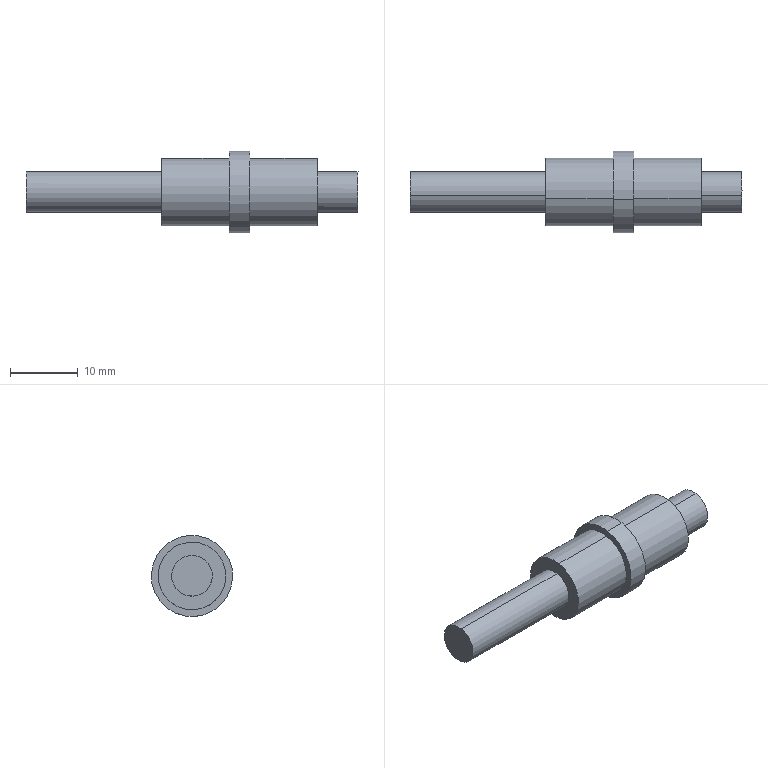Component | SolidWorks | GrippingMandrel-1 | 1 solid | 16 faces | box 49.01 x 12 x 12 mm | volume 2645 mm3 | cylinder 10 | plane 6 | commonest cylinder face diameters 6 x4 10 x4 12 x2
build123d program:
from build123d import *

# Parameters (mm, degrees)
SKETCH1_R           = 5
BOSS_EXTRUDE1_DEPTH = 10
SKETCH2_R           = 3
BOSS_EXTRUDE2_DEPTH = 6
SKETCH4_R           = 6
BOSS_EXTRUDE4_DEPTH = 3
SKETCH5_R           = 5
BOSS_EXTRUDE5_DEPTH = 10
BOSS_EXTRUDE6_START = 20
SKETCH6_R           = 3
BOSS_EXTRUDE6_DEPTH = 20


with BuildPart() as part:
    # Sketch1 → Boss-Extrude1 (new body)
    with BuildSketch(Plane(origin=(0, 0, 0), x_dir=(1, 0, 0), z_dir=(0, 1, 0))):
        with Locations(Location((0, 0, 0), (0, 0, 270))):
            Circle(SKETCH1_R)
    extrude(amount=BOSS_EXTRUDE1_DEPTH)

    # Sketch2 → Boss-Extrude2 (add)
    with BuildSketch(Plane(origin=(0, 0, 0), x_dir=(-1, 0, 0), z_dir=(0, -1, 0))):
        with Locations(Location((0, 0, 0), (0, 0, 90))):
            Circle(SKETCH2_R)
    extrude(amount=BOSS_EXTRUDE2_DEPTH)

    # Sketch4 → Boss-Extrude4 (add)
    with BuildSketch(Plane(origin=(0, 10, 0), x_dir=(1, 0, 0), z_dir=(0, 1, 0))):
        with Locations(Location((0, 0, 0), (0, 0, 270))):
            Circle(SKETCH4_R)
    extrude(amount=BOSS_EXTRUDE4_DEPTH)

    # Sketch5 → Boss-Extrude5 (add)
    with BuildSketch(Plane(origin=(0, 13, 0), x_dir=(1, 0, 0), z_dir=(0, 1, 0))):
        with Locations(Location((0, 0, 0), (0, 0, 270))):
            Circle(SKETCH5_R)
    extrude(amount=BOSS_EXTRUDE5_DEPTH)

    # Sketch6 → Boss-Extrude6 (add)
    with BuildSketch(Plane(origin=(0, 23, 0), x_dir=(1, 0, 0), z_dir=(0, 1, 0)).offset(BOSS_EXTRUDE6_START)):
        with Locations(Location((0, 0, 0), (0, 0, 90))):
            Circle(SKETCH6_R)
    extrude(amount=-BOSS_EXTRUDE6_DEPTH)


solid = part.part

# Placed as in the assembly
solid = solid.moved(Location((-104.642, 765.309, 1092.206), (-22.496, 0.05719, 90.024)))
STEP:
#1=CARTESIAN_POINT('',(-5.813,30.109,43.118));
#2=VERTEX_POINT('',#1);
#3=CARTESIAN_POINT('',(-5.813,30.152,42.886));
#4=VERTEX_POINT('',#3);
#5=CARTESIAN_POINT('',(-5.813,30.13,43.002));
#6=DIRECTION('',(-1.,-0.,0.00108));
#7=DIRECTION('',(0.001062,-0.1828,0.9831));
#8=AXIS2_PLACEMENT_3D('',#5,#6,#7);
#9=CIRCLE('',#8,0.1181);
#10=EDGE_CURVE('',#2,#4,#9,.T.);
#11=ORIENTED_EDGE('',*,*,#10,.F.);
#12=CARTESIAN_POINT('',(-5.025,30.109,43.117));
#13=VERTEX_POINT('',#12);
#14=CARTESIAN_POINT('',(-5.813,30.109,43.118));
#15=DIRECTION('',(1.,0.,-0.00108));
#16=VECTOR('',#15,39.37);
#17=LINE('',#14,#16);
#18=EDGE_CURVE('',#2,#13,#17,.T.);
#19=ORIENTED_EDGE('',*,*,#18,.T.);
#20=CARTESIAN_POINT('',(-5.025,30.152,42.885));
#21=VERTEX_POINT('',#20);
#22=CARTESIAN_POINT('',(-5.025,30.13,43.001));
#23=DIRECTION('',(-1.,-0.,0.00108));
#24=DIRECTION('',(0.001062,-0.1828,0.9831));
#25=AXIS2_PLACEMENT_3D('',#22,#23,#24);
#26=CIRCLE('',#25,0.1181);
#27=EDGE_CURVE('',#13,#21,#26,.T.);
#28=ORIENTED_EDGE('',*,*,#27,.T.);
#29=CARTESIAN_POINT('',(-5.813,30.152,42.886));
#30=DIRECTION('',(1.,0.,-0.00108));
#31=VECTOR('',#30,39.37);
#32=LINE('',#29,#31);
#33=EDGE_CURVE('',#4,#21,#32,.T.);
#34=ORIENTED_EDGE('',*,*,#33,.F.);
#35=EDGE_LOOP('',(#11,#19,#28,#34));
#36=FACE_OUTER_BOUND('',#35,.T.);
#37=CARTESIAN_POINT('',(-5.813,30.13,43.002));
#38=DIRECTION('',(1.,0.,-0.00108));
#39=DIRECTION('',(-0.001062,0.1828,-0.9831));
#40=AXIS2_PLACEMENT_3D('',#37,#38,#39);
#41=CYLINDRICAL_SURFACE('',#40,0.1181);
#42=ADVANCED_FACE('',(#36),#41,.T.);
#43=CARTESIAN_POINT('',(-5.025,30.094,43.195));
#44=VERTEX_POINT('',#43);
#45=CARTESIAN_POINT('',(-5.025,30.166,42.808));
#46=VERTEX_POINT('',#45);
#47=CARTESIAN_POINT('',(-5.025,30.13,43.001));
#48=DIRECTION('',(-1.,-0.,0.00108));
#49=DIRECTION('',(0.001062,-0.1828,0.9831));
#50=AXIS2_PLACEMENT_3D('',#47,#48,#49);
#51=CIRCLE('',#50,0.1969);
#52=EDGE_CURVE('',#44,#46,#51,.T.);
#53=ORIENTED_EDGE('',*,*,#52,.F.);
#54=CARTESIAN_POINT('',(-4.631,30.094,43.194));
#55=VERTEX_POINT('',#54);
#56=CARTESIAN_POINT('',(-5.025,30.094,43.195));
#57=DIRECTION('',(1.,0.,-0.00108));
#58=VECTOR('',#57,39.37);
#59=LINE('',#56,#58);
#60=EDGE_CURVE('',#44,#55,#59,.T.);
#61=ORIENTED_EDGE('',*,*,#60,.T.);
#62=CARTESIAN_POINT('',(-4.632,30.166,42.807));
#63=VERTEX_POINT('',#62);
#64=CARTESIAN_POINT('',(-4.632,30.13,43.001));
#65=DIRECTION('',(-1.,-0.,0.00108));
#66=DIRECTION('',(0.001062,-0.1828,0.9831));
#67=AXIS2_PLACEMENT_3D('',#64,#65,#66);
#68=CIRCLE('',#67,0.1969);
#69=EDGE_CURVE('',#55,#63,#68,.T.);
#70=ORIENTED_EDGE('',*,*,#69,.T.);
#71=CARTESIAN_POINT('',(-5.025,30.166,42.808));
#72=DIRECTION('',(1.,0.,-0.00108));
#73=VECTOR('',#72,39.37);
#74=LINE('',#71,#73);
#75=EDGE_CURVE('',#46,#63,#74,.T.);
#76=ORIENTED_EDGE('',*,*,#75,.F.);
#77=EDGE_LOOP('',(#53,#61,#70,#76));
#78=FACE_OUTER_BOUND('',#77,.T.);
#79=CARTESIAN_POINT('',(-5.025,30.13,43.001));
#80=DIRECTION('',(1.,0.,-0.00108));
#81=DIRECTION('',(-0.001062,0.1828,-0.9831));
#82=AXIS2_PLACEMENT_3D('',#79,#80,#81);
#83=CYLINDRICAL_SURFACE('',#82,0.1969);
#84=ADVANCED_FACE('',(#78),#83,.T.);
#85=CARTESIAN_POINT('',(-4.631,30.087,43.233));
#86=VERTEX_POINT('',#85);
#87=CARTESIAN_POINT('',(-4.632,30.173,42.769));
#88=VERTEX_POINT('',#87);
#89=CARTESIAN_POINT('',(-4.632,30.13,43.001));
#90=DIRECTION('',(-1.,-0.,0.00108));
#91=DIRECTION('',(0.001062,-0.1828,0.9831));
#92=AXIS2_PLACEMENT_3D('',#89,#90,#91);
#93=CIRCLE('',#92,0.2362);
#94=EDGE_CURVE('',#86,#88,#93,.T.);
#95=ORIENTED_EDGE('',*,*,#94,.F.);
#96=CARTESIAN_POINT('',(-4.513,30.087,43.233));
#97=VERTEX_POINT('',#96);
#98=CARTESIAN_POINT('',(-4.631,30.087,43.233));
#99=DIRECTION('',(1.,0.,-0.00108));
#100=VECTOR('',#99,39.37);
#101=LINE('',#98,#100);
#102=EDGE_CURVE('',#86,#97,#101,.T.);
#103=ORIENTED_EDGE('',*,*,#102,.T.);
#104=CARTESIAN_POINT('',(-4.514,30.173,42.768));
#105=VERTEX_POINT('',#104);
#106=CARTESIAN_POINT('',(-4.513,30.13,43.001));
#107=DIRECTION('',(-1.,-0.,0.00108));
#108=DIRECTION('',(0.001062,-0.1828,0.9831));
#109=AXIS2_PLACEMENT_3D('',#106,#107,#108);
#110=CIRCLE('',#109,0.2362);
#111=EDGE_CURVE('',#97,#105,#110,.T.);
#112=ORIENTED_EDGE('',*,*,#111,.T.);
#113=CARTESIAN_POINT('',(-4.632,30.173,42.769));
#114=DIRECTION('',(1.,0.,-0.00108));
#115=VECTOR('',#114,39.37);
#116=LINE('',#113,#115);
#117=EDGE_CURVE('',#88,#105,#116,.T.);
#118=ORIENTED_EDGE('',*,*,#117,.F.);
#119=EDGE_LOOP('',(#95,#103,#112,#118));
#120=FACE_OUTER_BOUND('',#119,.T.);
#121=CARTESIAN_POINT('',(-4.632,30.13,43.001));
#122=DIRECTION('',(1.,0.,-0.00108));
#123=DIRECTION('',(-0.001062,0.1828,-0.9831));
#124=AXIS2_PLACEMENT_3D('',#121,#122,#123);
#125=CYLINDRICAL_SURFACE('',#124,0.2362);
#126=ADVANCED_FACE('',(#120),#125,.T.);
#127=CARTESIAN_POINT('',(-3.884,30.152,42.884));
#128=VERTEX_POINT('',#127);
#129=CARTESIAN_POINT('',(-3.883,30.109,43.116));
#130=VERTEX_POINT('',#129);
#131=CARTESIAN_POINT('',(-3.884,30.13,43.));
#132=DIRECTION('',(1.,0.,-0.00108));
#133=DIRECTION('',(-0.001062,0.1828,-0.9831));
#134=AXIS2_PLACEMENT_3D('',#131,#132,#133);
#135=CIRCLE('',#134,0.1181);
#136=EDGE_CURVE('',#128,#130,#135,.T.);
#137=ORIENTED_EDGE('',*,*,#136,.F.);
#138=CARTESIAN_POINT('',(-4.12,30.152,42.884));
#139=VERTEX_POINT('',#138);
#140=CARTESIAN_POINT('',(-3.884,30.152,42.884));
#141=DIRECTION('',(-1.,-0.,0.00108));
#142=VECTOR('',#141,39.37);
#143=LINE('',#140,#142);
#144=EDGE_CURVE('',#128,#139,#143,.T.);
#145=ORIENTED_EDGE('',*,*,#144,.T.);
#146=CARTESIAN_POINT('',(-4.12,30.109,43.116));
#147=VERTEX_POINT('',#146);
#148=CARTESIAN_POINT('',(-4.12,30.13,43.));
#149=DIRECTION('',(1.,0.,-0.00108));
#150=DIRECTION('',(-0.001062,0.1828,-0.9831));
#151=AXIS2_PLACEMENT_3D('',#148,#149,#150);
#152=CIRCLE('',#151,0.1181);
#153=EDGE_CURVE('',#139,#147,#152,.T.);
#154=ORIENTED_EDGE('',*,*,#153,.T.);
#155=CARTESIAN_POINT('',(-3.883,30.109,43.116));
#156=DIRECTION('',(-1.,-0.,0.00108));
#157=VECTOR('',#156,39.37);
#158=LINE('',#155,#157);
#159=EDGE_CURVE('',#130,#147,#158,.T.);
#160=ORIENTED_EDGE('',*,*,#159,.F.);
#161=EDGE_LOOP('',(#137,#145,#154,#160));
#162=FACE_OUTER_BOUND('',#161,.T.);
#163=CARTESIAN_POINT('',(-3.884,30.13,43.));
#164=DIRECTION('',(-1.,-0.,0.00108));
#165=DIRECTION('',(0.001062,-0.1828,0.9831));
#166=AXIS2_PLACEMENT_3D('',#163,#164,#165);
#167=CYLINDRICAL_SURFACE('',#166,0.1181);
#168=ADVANCED_FACE('',(#162),#167,.T.);
#169=CARTESIAN_POINT('',(-4.513,30.094,43.194));
#170=VERTEX_POINT('',#169);
#171=CARTESIAN_POINT('',(-4.514,30.166,42.807));
#172=VERTEX_POINT('',#171);
#173=CARTESIAN_POINT('',(-4.513,30.13,43.001));
#174=DIRECTION('',(-1.,-0.,0.00108));
#175=DIRECTION('',(0.001062,-0.1828,0.9831));
#176=AXIS2_PLACEMENT_3D('',#173,#174,#175);
#177=CIRCLE('',#176,0.1969);
#178=EDGE_CURVE('',#170,#172,#177,.T.);
#179=ORIENTED_EDGE('',*,*,#178,.F.);
#180=CARTESIAN_POINT('',(-4.12,30.094,43.194));
#181=VERTEX_POINT('',#180);
#182=CARTESIAN_POINT('',(-4.513,30.094,43.194));
#183=DIRECTION('',(1.,0.,-0.00108));
#184=VECTOR('',#183,39.37);
#185=LINE('',#182,#184);
#186=EDGE_CURVE('',#170,#181,#185,.T.);
#187=ORIENTED_EDGE('',*,*,#186,.T.);
#188=CARTESIAN_POINT('',(-4.12,30.166,42.807));
#189=VERTEX_POINT('',#188);
#190=CARTESIAN_POINT('',(-4.12,30.13,43.));
#191=DIRECTION('',(-1.,-0.,0.00108));
#192=DIRECTION('',(0.001062,-0.1828,0.9831));
#193=AXIS2_PLACEMENT_3D('',#190,#191,#192);
#194=CIRCLE('',#193,0.1969);
#195=EDGE_CURVE('',#181,#189,#194,.T.);
#196=ORIENTED_EDGE('',*,*,#195,.T.);
#197=CARTESIAN_POINT('',(-4.514,30.166,42.807));
#198=DIRECTION('',(1.,0.,-0.00108));
#199=VECTOR('',#198,39.37);
#200=LINE('',#197,#199);
#201=EDGE_CURVE('',#172,#189,#200,.T.);
#202=ORIENTED_EDGE('',*,*,#201,.F.);
#203=EDGE_LOOP('',(#179,#187,#196,#202));
#204=FACE_OUTER_BOUND('',#203,.T.);
#205=CARTESIAN_POINT('',(-4.513,30.13,43.001));
#206=DIRECTION('',(1.,0.,-0.00108));
#207=DIRECTION('',(-0.001062,0.1828,-0.9831));
#208=AXIS2_PLACEMENT_3D('',#205,#206,#207);
#209=CYLINDRICAL_SURFACE('',#208,0.1969);
#210=ADVANCED_FACE('',(#204),#209,.T.);
#211=ORIENTED_EDGE('',*,*,#186,.F.);
#212=CARTESIAN_POINT('',(-4.513,30.13,43.001));
#213=DIRECTION('',(-1.,-0.,0.00108));
#214=DIRECTION('',(0.001062,-0.1828,0.9831));
#215=AXIS2_PLACEMENT_3D('',#212,#213,#214);
#216=CIRCLE('',#215,0.1969);
#217=EDGE_CURVE('',#172,#170,#216,.T.);
#218=ORIENTED_EDGE('',*,*,#217,.F.);
#219=ORIENTED_EDGE('',*,*,#201,.T.);
#220=CARTESIAN_POINT('',(-4.12,30.13,43.));
#221=DIRECTION('',(-1.,-0.,0.00108));
#222=DIRECTION('',(0.001062,-0.1828,0.9831));
#223=AXIS2_PLACEMENT_3D('',#220,#221,#222);
#224=CIRCLE('',#223,0.1969);
#225=EDGE_CURVE('',#189,#181,#224,.T.);
#226=ORIENTED_EDGE('',*,*,#225,.T.);
#227=EDGE_LOOP('',(#211,#218,#219,#226));
#228=FACE_OUTER_BOUND('',#227,.T.);
#229=CARTESIAN_POINT('',(-4.513,30.13,43.001));
#230=DIRECTION('',(1.,0.,-0.00108));
#231=DIRECTION('',(-0.001062,0.1828,-0.9831));
#232=AXIS2_PLACEMENT_3D('',#229,#230,#231);
#233=CYLINDRICAL_SURFACE('',#232,0.1969);
#234=ADVANCED_FACE('',(#228),#233,.T.);
#235=CARTESIAN_POINT('',(-4.12,30.13,43.));
#236=DIRECTION('',(1.,0.,-0.00108));
#237=DIRECTION('',(-0.001062,0.1828,-0.9831));
#238=AXIS2_PLACEMENT_3D('',#235,#236,#237);
#239=CIRCLE('',#238,0.1181);
#240=EDGE_CURVE('',#147,#139,#239,.T.);
#241=ORIENTED_EDGE('',*,*,#240,.F.);
#242=ORIENTED_EDGE('',*,*,#153,.F.);
#243=EDGE_LOOP('',(#241,#242));
#244=FACE_BOUND('',#243,.T.);
#245=ORIENTED_EDGE('',*,*,#225,.F.);
#246=ORIENTED_EDGE('',*,*,#195,.F.);
#247=EDGE_LOOP('',(#245,#246));
#248=FACE_OUTER_BOUND('',#247,.T.);
#249=CARTESIAN_POINT('',(-4.12,30.13,43.));
#250=DIRECTION('',(-1.,-0.,0.00108));
#251=DIRECTION('',(0.001062,-0.1828,0.9831));
#252=AXIS2_PLACEMENT_3D('',#249,#250,#251);
#253=PLANE('',#252);
#254=ADVANCED_FACE('',(#244,#248),#253,.F.);
#255=ORIENTED_EDGE('',*,*,#144,.F.);
#256=CARTESIAN_POINT('',(-3.884,30.13,43.));
#257=DIRECTION('',(1.,0.,-0.00108));
#258=DIRECTION('',(-0.001062,0.1828,-0.9831));
#259=AXIS2_PLACEMENT_3D('',#256,#257,#258);
#260=CIRCLE('',#259,0.1181);
#261=EDGE_CURVE('',#130,#128,#260,.T.);
#262=ORIENTED_EDGE('',*,*,#261,.F.);
#263=ORIENTED_EDGE('',*,*,#159,.T.);
#264=ORIENTED_EDGE('',*,*,#240,.T.);
#265=EDGE_LOOP('',(#255,#262,#263,#264));
#266=FACE_OUTER_BOUND('',#265,.T.);
#267=CARTESIAN_POINT('',(-3.884,30.13,43.));
#268=DIRECTION('',(-1.,-0.,0.00108));
#269=DIRECTION('',(0.001062,-0.1828,0.9831));
#270=AXIS2_PLACEMENT_3D('',#267,#268,#269);
#271=CYLINDRICAL_SURFACE('',#270,0.1181);
#272=ADVANCED_FACE('',(#266),#271,.T.);
#273=ORIENTED_EDGE('',*,*,#261,.T.);
#274=ORIENTED_EDGE('',*,*,#136,.T.);
#275=EDGE_LOOP('',(#273,#274));
#276=FACE_OUTER_BOUND('',#275,.T.);
#277=CARTESIAN_POINT('',(-3.884,30.13,43.));
#278=DIRECTION('',(1.,0.,-0.00108));
#279=DIRECTION('',(-0.001062,0.1828,-0.9831));
#280=AXIS2_PLACEMENT_3D('',#277,#278,#279);
#281=PLANE('',#280);
#282=ADVANCED_FACE('',(#276),#281,.T.);
#283=ORIENTED_EDGE('',*,*,#102,.F.);
#284=CARTESIAN_POINT('',(-4.632,30.13,43.001));
#285=DIRECTION('',(-1.,-0.,0.00108));
#286=DIRECTION('',(0.001062,-0.1828,0.9831));
#287=AXIS2_PLACEMENT_3D('',#284,#285,#286);
#288=CIRCLE('',#287,0.2362);
#289=EDGE_CURVE('',#88,#86,#288,.T.);
#290=ORIENTED_EDGE('',*,*,#289,.F.);
#291=ORIENTED_EDGE('',*,*,#117,.T.);
#292=CARTESIAN_POINT('',(-4.513,30.13,43.001));
#293=DIRECTION('',(-1.,-0.,0.00108));
#294=DIRECTION('',(0.001062,-0.1828,0.9831));
#295=AXIS2_PLACEMENT_3D('',#292,#293,#294);
#296=CIRCLE('',#295,0.2362);
#297=EDGE_CURVE('',#105,#97,#296,.T.);
#298=ORIENTED_EDGE('',*,*,#297,.T.);
#299=EDGE_LOOP('',(#283,#290,#291,#298));
#300=FACE_OUTER_BOUND('',#299,.T.);
#301=CARTESIAN_POINT('',(-4.632,30.13,43.001));
#302=DIRECTION('',(1.,0.,-0.00108));
#303=DIRECTION('',(-0.001062,0.1828,-0.9831));
#304=AXIS2_PLACEMENT_3D('',#301,#302,#303);
#305=CYLINDRICAL_SURFACE('',#304,0.2362);
#306=ADVANCED_FACE('',(#300),#305,.T.);
#307=CARTESIAN_POINT('',(-4.632,30.13,43.001));
#308=DIRECTION('',(-1.,-0.,0.00108));
#309=DIRECTION('',(0.001062,-0.1828,0.9831));
#310=AXIS2_PLACEMENT_3D('',#307,#308,#309);
#311=CIRCLE('',#310,0.1969);
#312=EDGE_CURVE('',#63,#55,#311,.T.);
#313=ORIENTED_EDGE('',*,*,#312,.F.);
#314=ORIENTED_EDGE('',*,*,#69,.F.);
#315=EDGE_LOOP('',(#313,#314));
#316=FACE_BOUND('',#315,.T.);
#317=ORIENTED_EDGE('',*,*,#289,.T.);
#318=ORIENTED_EDGE('',*,*,#94,.T.);
#319=EDGE_LOOP('',(#317,#318));
#320=FACE_OUTER_BOUND('',#319,.T.);
#321=CARTESIAN_POINT('',(-4.632,30.13,43.001));
#322=DIRECTION('',(-1.,-0.,0.00108));
#323=DIRECTION('',(0.001062,-0.1828,0.9831));
#324=AXIS2_PLACEMENT_3D('',#321,#322,#323);
#325=PLANE('',#324);
#326=ADVANCED_FACE('',(#316,#320),#325,.T.);
#327=ORIENTED_EDGE('',*,*,#217,.T.);
#328=ORIENTED_EDGE('',*,*,#178,.T.);
#329=EDGE_LOOP('',(#327,#328));
#330=FACE_BOUND('',#329,.T.);
#331=ORIENTED_EDGE('',*,*,#297,.F.);
#332=ORIENTED_EDGE('',*,*,#111,.F.);
#333=EDGE_LOOP('',(#331,#332));
#334=FACE_OUTER_BOUND('',#333,.T.);
#335=CARTESIAN_POINT('',(-4.513,30.13,43.001));
#336=DIRECTION('',(-1.,-0.,0.00108));
#337=DIRECTION('',(0.001062,-0.1828,0.9831));
#338=AXIS2_PLACEMENT_3D('',#335,#336,#337);
#339=PLANE('',#338);
#340=ADVANCED_FACE('',(#330,#334),#339,.F.);
#341=ORIENTED_EDGE('',*,*,#60,.F.);
#342=CARTESIAN_POINT('',(-5.025,30.13,43.001));
#343=DIRECTION('',(-1.,-0.,0.00108));
#344=DIRECTION('',(0.001062,-0.1828,0.9831));
#345=AXIS2_PLACEMENT_3D('',#342,#343,#344);
#346=CIRCLE('',#345,0.1969);
#347=EDGE_CURVE('',#46,#44,#346,.T.);
#348=ORIENTED_EDGE('',*,*,#347,.F.);
#349=ORIENTED_EDGE('',*,*,#75,.T.);
#350=ORIENTED_EDGE('',*,*,#312,.T.);
#351=EDGE_LOOP('',(#341,#348,#349,#350));
#352=FACE_OUTER_BOUND('',#351,.T.);
#353=CARTESIAN_POINT('',(-5.025,30.13,43.001));
#354=DIRECTION('',(1.,0.,-0.00108));
#355=DIRECTION('',(-0.001062,0.1828,-0.9831));
#356=AXIS2_PLACEMENT_3D('',#353,#354,#355);
#357=CYLINDRICAL_SURFACE('',#356,0.1969);
#358=ADVANCED_FACE('',(#352),#357,.T.);
#359=CARTESIAN_POINT('',(-5.025,30.13,43.001));
#360=DIRECTION('',(-1.,-0.,0.00108));
#361=DIRECTION('',(0.001062,-0.1828,0.9831));
#362=AXIS2_PLACEMENT_3D('',#359,#360,#361);
#363=CIRCLE('',#362,0.1181);
#364=EDGE_CURVE('',#21,#13,#363,.T.);
#365=ORIENTED_EDGE('',*,*,#364,.F.);
#366=ORIENTED_EDGE('',*,*,#27,.F.);
#367=EDGE_LOOP('',(#365,#366));
#368=FACE_BOUND('',#367,.T.);
#369=ORIENTED_EDGE('',*,*,#347,.T.);
#370=ORIENTED_EDGE('',*,*,#52,.T.);
#371=EDGE_LOOP('',(#369,#370));
#372=FACE_OUTER_BOUND('',#371,.T.);
#373=CARTESIAN_POINT('',(-5.025,30.13,43.001));
#374=DIRECTION('',(-1.,-0.,0.00108));
#375=DIRECTION('',(0.001062,-0.1828,0.9831));
#376=AXIS2_PLACEMENT_3D('',#373,#374,#375);
#377=PLANE('',#376);
#378=ADVANCED_FACE('',(#368,#372),#377,.T.);
#379=ORIENTED_EDGE('',*,*,#18,.F.);
#380=CARTESIAN_POINT('',(-5.813,30.13,43.002));
#381=DIRECTION('',(-1.,-0.,0.00108));
#382=DIRECTION('',(0.001062,-0.1828,0.9831));
#383=AXIS2_PLACEMENT_3D('',#380,#381,#382);
#384=CIRCLE('',#383,0.1181);
#385=EDGE_CURVE('',#4,#2,#384,.T.);
#386=ORIENTED_EDGE('',*,*,#385,.F.);
#387=ORIENTED_EDGE('',*,*,#33,.T.);
#388=ORIENTED_EDGE('',*,*,#364,.T.);
#389=EDGE_LOOP('',(#379,#386,#387,#388));
#390=FACE_OUTER_BOUND('',#389,.T.);
#391=CARTESIAN_POINT('',(-5.813,30.13,43.002));
#392=DIRECTION('',(1.,0.,-0.00108));
#393=DIRECTION('',(-0.001062,0.1828,-0.9831));
#394=AXIS2_PLACEMENT_3D('',#391,#392,#393);
#395=CYLINDRICAL_SURFACE('',#394,0.1181);
#396=ADVANCED_FACE('',(#390),#395,.T.);
#397=ORIENTED_EDGE('',*,*,#385,.T.);
#398=ORIENTED_EDGE('',*,*,#10,.T.);
#399=EDGE_LOOP('',(#397,#398));
#400=FACE_OUTER_BOUND('',#399,.T.);
#401=CARTESIAN_POINT('',(-5.813,30.13,43.002));
#402=DIRECTION('',(-1.,-0.,0.00108));
#403=DIRECTION('',(0.001062,-0.1828,0.9831));
#404=AXIS2_PLACEMENT_3D('',#401,#402,#403);
#405=PLANE('',#404);
#406=ADVANCED_FACE('',(#400),#405,.T.);
#407=CLOSED_SHELL('',(#42,#84,#126,#168,#210,#234,#254,#272,#282,#306,#326,#340,#358,#378,#396,#406));
#408=MANIFOLD_SOLID_BREP('',#407);
#409=CARTESIAN_POINT('',(0.,0.,0.));
#410=DIRECTION('',(0.,0.,1.));
#411=DIRECTION('',(1.,0.,0.));
#412=AXIS2_PLACEMENT_3D('',#409,#410,#411);
#413=(LENGTH_UNIT()NAMED_UNIT(*)SI_UNIT($,.METRE.));
#414=LENGTH_MEASURE_WITH_UNIT(LENGTH_MEASURE(0.0254),#413);
#415=DIMENSIONAL_EXPONENTS(1.,0.,0.,0.,0.,0.,0.);
#416=(CONVERSION_BASED_UNIT('',#414)LENGTH_UNIT()NAMED_UNIT(#415));
#417=UNCERTAINTY_MEASURE_WITH_UNIT(LENGTH_MEASURE(0.00001),#416,'','');
#418=(NAMED_UNIT(*)PLANE_ANGLE_UNIT()SI_UNIT($,.RADIAN.));
#419=(NAMED_UNIT(*)SI_UNIT($,.STERADIAN.)SOLID_ANGLE_UNIT());
#420=(GEOMETRIC_REPRESENTATION_CONTEXT(3)GLOBAL_UNCERTAINTY_ASSIGNED_CONTEXT((#417))GLOBAL_UNIT_ASSIGNED_CONTEXT((#416,#418,#419))REPRESENTATION_CONTEXT('',''));
#421=ADVANCED_BREP_SHAPE_REPRESENTATION('',(#408,#412),#420);
#422=COLOUR_RGB('',0.7922,0.8196,0.9333);
#423=FILL_AREA_STYLE_COLOUR('',#422);
#424=FILL_AREA_STYLE('',(#423));
#425=SURFACE_STYLE_FILL_AREA(#424);
#426=SURFACE_SIDE_STYLE('',(#425));
#427=SURFACE_STYLE_USAGE(.BOTH.,#426);
#428=PRESENTATION_STYLE_ASSIGNMENT((#427));
#429=STYLED_ITEM('',(#428),#408);
#430=PRESENTATION_LAYER_ASSIGNMENT('','',(#429));
#431=(LENGTH_UNIT()NAMED_UNIT(*)SI_UNIT($,.METRE.));
#432=LENGTH_MEASURE_WITH_UNIT(LENGTH_MEASURE(0.0254),#431);
#433=DIMENSIONAL_EXPONENTS(1.,0.,0.,0.,0.,0.,0.);
#434=(CONVERSION_BASED_UNIT('',#432)LENGTH_UNIT()NAMED_UNIT(#433));
#435=UNCERTAINTY_MEASURE_WITH_UNIT(LENGTH_MEASURE(0.00001),#434,'','');
#436=(NAMED_UNIT(*)PLANE_ANGLE_UNIT()SI_UNIT($,.RADIAN.));
#437=(NAMED_UNIT(*)SI_UNIT($,.STERADIAN.)SOLID_ANGLE_UNIT());
#438=(GEOMETRIC_REPRESENTATION_CONTEXT(3)GLOBAL_UNCERTAINTY_ASSIGNED_CONTEXT((#435))GLOBAL_UNIT_ASSIGNED_CONTEXT((#434,#436,#437))REPRESENTATION_CONTEXT('',''));
#439=MECHANICAL_DESIGN_GEOMETRIC_PRESENTATION_REPRESENTATION('',(#429),#438);